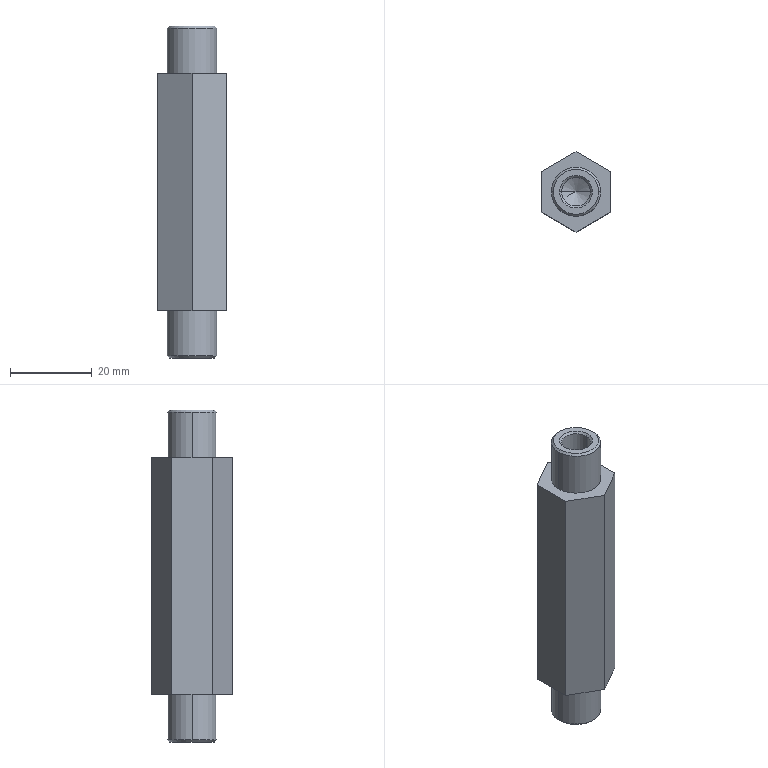Component | SolidWorks | YX-04-102GluePaperFeedingColumn-2 | 1 solid | 30 faces | box 17 x 19.63 x 81 mm | volume 15432 mm3 | cone 12 | plane 10 | cylinder 8 | commonest cylinder face diameters 7 x4 12 x4 | material Brass
build123d program:
from build123d import *

# Parameters (mm, degrees)
BOSS_EXTRUDE1_DEPTH          = 58
SKETCH2_W                    = 11.5
SKETCH2_H                    = 6
SKETCH3_W                    = 11.5
SKETCH3_H                    = 6
F_7_0_7_DIAMETER_HOLE1_D     = 7
F_7_0_7_DIAMETER_HOLE1_DEPTH = 21
F_7_0_7_DIAMETER_HOLE1_TIP   = 2.103
F_7_0_7_DIAMETER_HOLE2_D     = 7
F_7_0_7_DIAMETER_HOLE2_DEPTH = 21
F_7_0_7_DIAMETER_HOLE2_TIP   = 2.103
CHAMFER1_SIZE                = 0.5


with BuildPart() as part:
    # Sketch1 → Boss-Extrude1 (new body)
    with BuildSketch(Plane(origin=(29, 0, 0), x_dir=(0, 0, -1), z_dir=(1, 0, 0))):
        Polygon((8.5, -4.907), (8.5, 4.907), (0, 9.815), (-8.5, 4.907), (-8.5, -4.907), (0, -9.815), align=None)
    extrude(amount=-BOSS_EXTRUDE1_DEPTH)

    # Sketch2 → Revolve1 (revolve)
    with BuildSketch(Plane.XY, mode=Mode.PRIVATE) as revolve1_sk:
        with Locations((-34.75, 3)):
            Rectangle(SKETCH2_W, SKETCH2_H)
    revolve(revolve1_sk.sketch.rotate(Axis((-40.5, 0, 0), (1, 0, 0)), 270), axis=Axis((-40.5, 0, 0), (1, 0, 0)))

    # Sketch3 → Revolve2 (revolve)
    with BuildSketch(Plane.XY, mode=Mode.PRIVATE) as revolve2_sk:
        with Locations((34.75, 3)):
            Rectangle(SKETCH3_W, SKETCH3_H)
    revolve(revolve2_sk.sketch.rotate(Axis((29, 0, 0), (1, 0, 0)), 270), axis=Axis((29, 0, 0), (1, 0, 0)))

    # 7.0 _7_ Diameter Hole1
    with Locations(Plane.ZY.offset(40.5)):
        with Locations((0, 0)):
            Hole(F_7_0_7_DIAMETER_HOLE1_D / 2, depth=F_7_0_7_DIAMETER_HOLE1_DEPTH)
            with Locations((0, 0, -(F_7_0_7_DIAMETER_HOLE1_DEPTH + F_7_0_7_DIAMETER_HOLE1_TIP / 2))):  # 118° drill point
                Cone(0, F_7_0_7_DIAMETER_HOLE1_D / 2, F_7_0_7_DIAMETER_HOLE1_TIP, mode=Mode.SUBTRACT)

    # 7.0 _7_ Diameter Hole2
    with Locations(Plane(origin=(40.5, 0, 0), x_dir=(0, 0, -1), z_dir=(1, 0, 0))):
        with Locations((0, 0)):
            Hole(F_7_0_7_DIAMETER_HOLE2_D / 2, depth=F_7_0_7_DIAMETER_HOLE2_DEPTH)
            with Locations((0, 0, -(F_7_0_7_DIAMETER_HOLE2_DEPTH + F_7_0_7_DIAMETER_HOLE2_TIP / 2))):  # 118° drill point
                Cone(0, F_7_0_7_DIAMETER_HOLE2_D / 2, F_7_0_7_DIAMETER_HOLE2_TIP, mode=Mode.SUBTRACT)

    # Chamfer1
    chamfer1_edges = [part.edges().sort_by_distance(p)[0] for p in [
        (-40.5, 0, 6),
        (40.5, 0, 6),
        (-40.5, 0, 3.5),
        (40.5, 0, -3.5),
    ]]
    chamfer(chamfer1_edges, length=CHAMFER1_SIZE)


solid = part.part

# Placed as in the assembly
solid = solid.moved(Location((-123.397, 46.262, 235), (0, 90, 0)))
STEP:
#1=COLOUR_RGB('',0.7922,0.8196,0.9333);
#2=FILL_AREA_STYLE_COLOUR('',#1);
#3=FILL_AREA_STYLE('',(#2));
#4=SURFACE_STYLE_FILL_AREA(#3);
#5=SURFACE_SIDE_STYLE('',(#4));
#6=SURFACE_STYLE_USAGE(.BOTH.,#5);
#7=PRESENTATION_STYLE_ASSIGNMENT((#6));
#8=CARTESIAN_POINT('',(-4.72,1.821,7.677));
#9=VERTEX_POINT('',#8);
#10=CARTESIAN_POINT('',(-4.996,1.821,7.677));
#11=VERTEX_POINT('',#10);
#12=CARTESIAN_POINT('',(-4.858,1.821,7.677));
#13=DIRECTION('',(0.,0.,-1.));
#14=DIRECTION('',(-1.,0.,0.));
#15=AXIS2_PLACEMENT_3D('',#12,#13,#14);
#16=CIRCLE('',#15,0.1378);
#17=EDGE_CURVE('',#9,#11,#16,.T.);
#18=ORIENTED_EDGE('',*,*,#17,.F.);
#19=CARTESIAN_POINT('',(-4.701,1.821,7.657));
#20=VERTEX_POINT('',#19);
#21=CARTESIAN_POINT('',(-4.72,1.821,7.677));
#22=DIRECTION('',(0.7071,0.,-0.7071));
#23=VECTOR('',#22,39.37);
#24=LINE('',#21,#23);
#25=EDGE_CURVE('',#9,#20,#24,.T.);
#26=ORIENTED_EDGE('',*,*,#25,.T.);
#27=CARTESIAN_POINT('',(-5.016,1.821,7.657));
#28=VERTEX_POINT('',#27);
#29=CARTESIAN_POINT('',(-4.858,1.821,7.657));
#30=DIRECTION('',(0.,0.,1.));
#31=DIRECTION('',(-1.,0.,0.));
#32=AXIS2_PLACEMENT_3D('',#29,#30,#31);
#33=CIRCLE('',#32,0.1575);
#34=EDGE_CURVE('',#28,#20,#33,.T.);
#35=ORIENTED_EDGE('',*,*,#34,.F.);
#36=CARTESIAN_POINT('',(-4.996,1.821,7.677));
#37=DIRECTION('',(-0.7071,0.,-0.7071));
#38=VECTOR('',#37,39.37);
#39=LINE('',#36,#38);
#40=EDGE_CURVE('',#11,#28,#39,.T.);
#41=ORIENTED_EDGE('',*,*,#40,.F.);
#42=EDGE_LOOP('',(#18,#26,#35,#41));
#43=FACE_OUTER_BOUND('',#42,.T.);
#44=CARTESIAN_POINT('',(-4.858,1.821,7.677));
#45=DIRECTION('',(0.,0.,-1.));
#46=DIRECTION('',(-1.,0.,0.));
#47=AXIS2_PLACEMENT_3D('',#44,#45,#46);
#48=CONICAL_SURFACE('',#47,0.1378,0.7854);
#49=ADVANCED_FACE('',(#43),#48,.F.);
#50=CARTESIAN_POINT('',(-4.996,1.821,10.827));
#51=VERTEX_POINT('',#50);
#52=CARTESIAN_POINT('',(-4.72,1.821,10.827));
#53=VERTEX_POINT('',#52);
#54=CARTESIAN_POINT('',(-4.858,1.821,10.827));
#55=DIRECTION('',(0.,0.,1.));
#56=DIRECTION('',(1.,0.,0.));
#57=AXIS2_PLACEMENT_3D('',#54,#55,#56);
#58=CIRCLE('',#57,0.1378);
#59=EDGE_CURVE('',#51,#53,#58,.T.);
#60=ORIENTED_EDGE('',*,*,#59,.F.);
#61=CARTESIAN_POINT('',(-5.016,1.821,10.846));
#62=VERTEX_POINT('',#61);
#63=CARTESIAN_POINT('',(-4.996,1.821,10.827));
#64=DIRECTION('',(-0.7071,0.,0.7071));
#65=VECTOR('',#64,39.37);
#66=LINE('',#63,#65);
#67=EDGE_CURVE('',#51,#62,#66,.T.);
#68=ORIENTED_EDGE('',*,*,#67,.T.);
#69=CARTESIAN_POINT('',(-4.701,1.821,10.846));
#70=VERTEX_POINT('',#69);
#71=CARTESIAN_POINT('',(-4.858,1.821,10.846));
#72=DIRECTION('',(0.,0.,-1.));
#73=DIRECTION('',(1.,0.,0.));
#74=AXIS2_PLACEMENT_3D('',#71,#72,#73);
#75=CIRCLE('',#74,0.1575);
#76=EDGE_CURVE('',#70,#62,#75,.T.);
#77=ORIENTED_EDGE('',*,*,#76,.F.);
#78=CARTESIAN_POINT('',(-4.72,1.821,10.827));
#79=DIRECTION('',(0.7071,0.,0.7071));
#80=VECTOR('',#79,39.37);
#81=LINE('',#78,#80);
#82=EDGE_CURVE('',#53,#70,#81,.T.);
#83=ORIENTED_EDGE('',*,*,#82,.F.);
#84=EDGE_LOOP('',(#60,#68,#77,#83));
#85=FACE_OUTER_BOUND('',#84,.T.);
#86=CARTESIAN_POINT('',(-4.858,1.821,10.827));
#87=DIRECTION('',(0.,0.,1.));
#88=DIRECTION('',(1.,0.,0.));
#89=AXIS2_PLACEMENT_3D('',#86,#87,#88);
#90=CONICAL_SURFACE('',#89,0.1378,0.7854);
#91=ADVANCED_FACE('',(#85),#90,.F.);
#92=CARTESIAN_POINT('',(-4.642,1.821,10.846));
#93=VERTEX_POINT('',#92);
#94=CARTESIAN_POINT('',(-5.075,1.821,10.846));
#95=VERTEX_POINT('',#94);
#96=CARTESIAN_POINT('',(-4.858,1.821,10.846));
#97=DIRECTION('',(0.,0.,1.));
#98=DIRECTION('',(1.,0.,0.));
#99=AXIS2_PLACEMENT_3D('',#96,#97,#98);
#100=CIRCLE('',#99,0.2165);
#101=EDGE_CURVE('',#93,#95,#100,.T.);
#102=ORIENTED_EDGE('',*,*,#101,.F.);
#103=CARTESIAN_POINT('',(-4.622,1.821,10.827));
#104=VERTEX_POINT('',#103);
#105=CARTESIAN_POINT('',(-4.642,1.821,10.846));
#106=DIRECTION('',(0.7071,0.,-0.7071));
#107=VECTOR('',#106,39.37);
#108=LINE('',#105,#107);
#109=EDGE_CURVE('',#93,#104,#108,.T.);
#110=ORIENTED_EDGE('',*,*,#109,.T.);
#111=CARTESIAN_POINT('',(-5.094,1.821,10.827));
#112=VERTEX_POINT('',#111);
#113=CARTESIAN_POINT('',(-4.858,1.821,10.827));
#114=DIRECTION('',(0.,0.,-1.));
#115=DIRECTION('',(1.,0.,0.));
#116=AXIS2_PLACEMENT_3D('',#113,#114,#115);
#117=CIRCLE('',#116,0.2362);
#118=EDGE_CURVE('',#112,#104,#117,.T.);
#119=ORIENTED_EDGE('',*,*,#118,.F.);
#120=CARTESIAN_POINT('',(-5.075,1.821,10.846));
#121=DIRECTION('',(-0.7071,0.,-0.7071));
#122=VECTOR('',#121,39.37);
#123=LINE('',#120,#122);
#124=EDGE_CURVE('',#95,#112,#123,.T.);
#125=ORIENTED_EDGE('',*,*,#124,.F.);
#126=EDGE_LOOP('',(#102,#110,#119,#125));
#127=FACE_OUTER_BOUND('',#126,.T.);
#128=CARTESIAN_POINT('',(-4.858,1.821,10.846));
#129=DIRECTION('',(0.,0.,-1.));
#130=DIRECTION('',(-1.,0.,0.));
#131=AXIS2_PLACEMENT_3D('',#128,#129,#130);
#132=CONICAL_SURFACE('',#131,0.2165,0.7854);
#133=ADVANCED_FACE('',(#127),#132,.T.);
#134=CARTESIAN_POINT('',(-5.075,1.821,7.657));
#135=VERTEX_POINT('',#134);
#136=CARTESIAN_POINT('',(-4.642,1.821,7.657));
#137=VERTEX_POINT('',#136);
#138=CARTESIAN_POINT('',(-4.858,1.821,7.657));
#139=DIRECTION('',(0.,0.,-1.));
#140=DIRECTION('',(-1.,0.,0.));
#141=AXIS2_PLACEMENT_3D('',#138,#139,#140);
#142=CIRCLE('',#141,0.2165);
#143=EDGE_CURVE('',#135,#137,#142,.T.);
#144=ORIENTED_EDGE('',*,*,#143,.F.);
#145=CARTESIAN_POINT('',(-5.094,1.821,7.677));
#146=VERTEX_POINT('',#145);
#147=CARTESIAN_POINT('',(-5.094,1.821,7.677));
#148=DIRECTION('',(-0.7071,0.,0.7071));
#149=VECTOR('',#148,39.37);
#150=LINE('',#147,#149);
#151=EDGE_CURVE('',#135,#146,#150,.T.);
#152=ORIENTED_EDGE('',*,*,#151,.T.);
#153=CARTESIAN_POINT('',(-4.622,1.821,7.677));
#154=VERTEX_POINT('',#153);
#155=CARTESIAN_POINT('',(-4.858,1.821,7.677));
#156=DIRECTION('',(0.,0.,1.));
#157=DIRECTION('',(-1.,0.,0.));
#158=AXIS2_PLACEMENT_3D('',#155,#156,#157);
#159=CIRCLE('',#158,0.2362);
#160=EDGE_CURVE('',#154,#146,#159,.T.);
#161=ORIENTED_EDGE('',*,*,#160,.F.);
#162=CARTESIAN_POINT('',(-4.622,1.821,7.677));
#163=DIRECTION('',(0.7071,0.,0.7071));
#164=VECTOR('',#163,39.37);
#165=LINE('',#162,#164);
#166=EDGE_CURVE('',#137,#154,#165,.T.);
#167=ORIENTED_EDGE('',*,*,#166,.F.);
#168=EDGE_LOOP('',(#144,#152,#161,#167));
#169=FACE_OUTER_BOUND('',#168,.T.);
#170=CARTESIAN_POINT('',(-4.858,1.821,7.677));
#171=DIRECTION('',(0.,0.,1.));
#172=DIRECTION('',(1.,0.,0.));
#173=AXIS2_PLACEMENT_3D('',#170,#171,#172);
#174=CONICAL_SURFACE('',#173,0.2362,0.7854);
#175=ADVANCED_FACE('',(#169),#174,.T.);
#176=CARTESIAN_POINT('',(-4.996,1.821,10.02));
#177=VERTEX_POINT('',#176);
#178=CARTESIAN_POINT('',(-4.72,1.821,10.02));
#179=VERTEX_POINT('',#178);
#180=CARTESIAN_POINT('',(-4.858,1.821,10.02));
#181=DIRECTION('',(0.,0.,1.));
#182=DIRECTION('',(1.,0.,0.));
#183=AXIS2_PLACEMENT_3D('',#180,#181,#182);
#184=CIRCLE('',#183,0.1378);
#185=EDGE_CURVE('',#177,#179,#184,.T.);
#186=ORIENTED_EDGE('',*,*,#185,.F.);
#187=CARTESIAN_POINT('',(-4.996,1.821,10.846));
#188=DIRECTION('',(0.,0.,1.));
#189=VECTOR('',#188,39.37);
#190=LINE('',#187,#189);
#191=EDGE_CURVE('',#177,#51,#190,.T.);
#192=ORIENTED_EDGE('',*,*,#191,.T.);
#193=ORIENTED_EDGE('',*,*,#59,.T.);
#194=CARTESIAN_POINT('',(-4.72,1.821,10.846));
#195=DIRECTION('',(0.,0.,1.));
#196=VECTOR('',#195,39.37);
#197=LINE('',#194,#196);
#198=EDGE_CURVE('',#179,#53,#197,.T.);
#199=ORIENTED_EDGE('',*,*,#198,.F.);
#200=EDGE_LOOP('',(#186,#192,#193,#199));
#201=FACE_OUTER_BOUND('',#200,.T.);
#202=CARTESIAN_POINT('',(-4.858,1.821,10.846));
#203=DIRECTION('',(0.,0.,1.));
#204=DIRECTION('',(1.,0.,0.));
#205=AXIS2_PLACEMENT_3D('',#202,#203,#204);
#206=CYLINDRICAL_SURFACE('',#205,0.1378);
#207=ADVANCED_FACE('',(#201),#206,.F.);
#208=CARTESIAN_POINT('',(-4.858,1.821,9.937));
#209=VERTEX_POINT('',#208);
#210=CARTESIAN_POINT('',(-4.72,1.821,10.02));
#211=DIRECTION('',(0.8572,0.,0.515));
#212=VECTOR('',#211,39.37);
#213=LINE('',#210,#212);
#214=EDGE_CURVE('',#209,#179,#213,.T.);
#215=ORIENTED_EDGE('',*,*,#214,.F.);
#216=CARTESIAN_POINT('',(-4.996,1.821,10.02));
#217=DIRECTION('',(-0.8572,0.,0.515));
#218=VECTOR('',#217,39.37);
#219=LINE('',#216,#218);
#220=EDGE_CURVE('',#209,#177,#219,.T.);
#221=ORIENTED_EDGE('',*,*,#220,.T.);
#222=ORIENTED_EDGE('',*,*,#185,.T.);
#223=EDGE_LOOP('',(#215,#221,#222));
#224=FACE_OUTER_BOUND('',#223,.T.);
#225=CARTESIAN_POINT('',(-4.858,1.821,10.02));
#226=DIRECTION('',(0.,0.,1.));
#227=DIRECTION('',(1.,0.,0.));
#228=AXIS2_PLACEMENT_3D('',#225,#226,#227);
#229=CONICAL_SURFACE('',#228,0.1378,1.03);
#230=ADVANCED_FACE('',(#224),#229,.F.);
#231=CARTESIAN_POINT('',(-4.72,1.821,8.484));
#232=VERTEX_POINT('',#231);
#233=CARTESIAN_POINT('',(-4.996,1.821,8.484));
#234=VERTEX_POINT('',#233);
#235=CARTESIAN_POINT('',(-4.858,1.821,8.484));
#236=DIRECTION('',(0.,0.,-1.));
#237=DIRECTION('',(-1.,0.,0.));
#238=AXIS2_PLACEMENT_3D('',#235,#236,#237);
#239=CIRCLE('',#238,0.1378);
#240=EDGE_CURVE('',#232,#234,#239,.T.);
#241=ORIENTED_EDGE('',*,*,#240,.F.);
#242=CARTESIAN_POINT('',(-4.72,1.821,7.657));
#243=DIRECTION('',(0.,0.,-1.));
#244=VECTOR('',#243,39.37);
#245=LINE('',#242,#244);
#246=EDGE_CURVE('',#232,#9,#245,.T.);
#247=ORIENTED_EDGE('',*,*,#246,.T.);
#248=ORIENTED_EDGE('',*,*,#17,.T.);
#249=CARTESIAN_POINT('',(-4.996,1.821,7.657));
#250=DIRECTION('',(0.,0.,-1.));
#251=VECTOR('',#250,39.37);
#252=LINE('',#249,#251);
#253=EDGE_CURVE('',#234,#11,#252,.T.);
#254=ORIENTED_EDGE('',*,*,#253,.F.);
#255=EDGE_LOOP('',(#241,#247,#248,#254));
#256=FACE_OUTER_BOUND('',#255,.T.);
#257=CARTESIAN_POINT('',(-4.858,1.821,7.657));
#258=DIRECTION('',(0.,0.,-1.));
#259=DIRECTION('',(-1.,0.,0.));
#260=AXIS2_PLACEMENT_3D('',#257,#258,#259);
#261=CYLINDRICAL_SURFACE('',#260,0.1378);
#262=ADVANCED_FACE('',(#256),#261,.F.);
#263=CARTESIAN_POINT('',(-4.858,1.821,8.567));
#264=VERTEX_POINT('',#263);
#265=CARTESIAN_POINT('',(-4.996,1.821,8.484));
#266=DIRECTION('',(-0.8572,0.,-0.515));
#267=VECTOR('',#266,39.37);
#268=LINE('',#265,#267);
#269=EDGE_CURVE('',#264,#234,#268,.T.);
#270=ORIENTED_EDGE('',*,*,#269,.F.);
#271=CARTESIAN_POINT('',(-4.72,1.821,8.484));
#272=DIRECTION('',(0.8572,0.,-0.515));
#273=VECTOR('',#272,39.37);
#274=LINE('',#271,#273);
#275=EDGE_CURVE('',#264,#232,#274,.T.);
#276=ORIENTED_EDGE('',*,*,#275,.T.);
#277=ORIENTED_EDGE('',*,*,#240,.T.);
#278=EDGE_LOOP('',(#270,#276,#277));
#279=FACE_OUTER_BOUND('',#278,.T.);
#280=CARTESIAN_POINT('',(-4.858,1.821,8.484));
#281=DIRECTION('',(0.,0.,-1.));
#282=DIRECTION('',(-1.,0.,0.));
#283=AXIS2_PLACEMENT_3D('',#280,#281,#282);
#284=CONICAL_SURFACE('',#283,0.1378,1.03);
#285=ADVANCED_FACE('',(#279),#284,.F.);
#286=CARTESIAN_POINT('',(-4.622,1.821,10.394));
#287=VERTEX_POINT('',#286);
#288=CARTESIAN_POINT('',(-5.094,1.821,10.394));
#289=VERTEX_POINT('',#288);
#290=CARTESIAN_POINT('',(-4.858,1.821,10.394));
#291=DIRECTION('',(0.,0.,1.));
#292=DIRECTION('',(1.,0.,0.));
#293=AXIS2_PLACEMENT_3D('',#290,#291,#292);
#294=CIRCLE('',#293,0.2362);
#295=EDGE_CURVE('',#287,#289,#294,.T.);
#296=ORIENTED_EDGE('',*,*,#295,.T.);
#297=CARTESIAN_POINT('',(-5.094,1.821,10.394));
#298=DIRECTION('',(0.,0.,1.));
#299=VECTOR('',#298,39.37);
#300=LINE('',#297,#299);
#301=EDGE_CURVE('',#289,#112,#300,.T.);
#302=ORIENTED_EDGE('',*,*,#301,.T.);
#303=ORIENTED_EDGE('',*,*,#118,.T.);
#304=CARTESIAN_POINT('',(-4.622,1.821,10.394));
#305=DIRECTION('',(0.,0.,1.));
#306=VECTOR('',#305,39.37);
#307=LINE('',#304,#306);
#308=EDGE_CURVE('',#287,#104,#307,.T.);
#309=ORIENTED_EDGE('',*,*,#308,.F.);
#310=EDGE_LOOP('',(#296,#302,#303,#309));
#311=FACE_OUTER_BOUND('',#310,.T.);
#312=CARTESIAN_POINT('',(-4.858,1.821,10.394));
#313=DIRECTION('',(0.,0.,1.));
#314=DIRECTION('',(1.,0.,0.));
#315=AXIS2_PLACEMENT_3D('',#312,#313,#314);
#316=CYLINDRICAL_SURFACE('',#315,0.2362);
#317=ADVANCED_FACE('',(#311),#316,.T.);
#318=ORIENTED_EDGE('',*,*,#160,.T.);
#319=CARTESIAN_POINT('',(-5.094,1.821,8.11));
#320=VERTEX_POINT('',#319);
#321=CARTESIAN_POINT('',(-5.094,1.821,7.657));
#322=DIRECTION('',(0.,0.,1.));
#323=VECTOR('',#322,39.37);
#324=LINE('',#321,#323);
#325=EDGE_CURVE('',#146,#320,#324,.T.);
#326=ORIENTED_EDGE('',*,*,#325,.T.);
#327=CARTESIAN_POINT('',(-4.622,1.821,8.11));
#328=VERTEX_POINT('',#327);
#329=CARTESIAN_POINT('',(-4.858,1.821,8.11));
#330=DIRECTION('',(0.,0.,1.));
#331=DIRECTION('',(1.,0.,0.));
#332=AXIS2_PLACEMENT_3D('',#329,#330,#331);
#333=CIRCLE('',#332,0.2362);
#334=EDGE_CURVE('',#328,#320,#333,.T.);
#335=ORIENTED_EDGE('',*,*,#334,.F.);
#336=CARTESIAN_POINT('',(-4.622,1.821,7.657));
#337=DIRECTION('',(0.,0.,1.));
#338=VECTOR('',#337,39.37);
#339=LINE('',#336,#338);
#340=EDGE_CURVE('',#154,#328,#339,.T.);
#341=ORIENTED_EDGE('',*,*,#340,.F.);
#342=EDGE_LOOP('',(#318,#326,#335,#341));
#343=FACE_OUTER_BOUND('',#342,.T.);
#344=CARTESIAN_POINT('',(-4.858,1.821,7.657));
#345=DIRECTION('',(0.,0.,1.));
#346=DIRECTION('',(1.,0.,0.));
#347=AXIS2_PLACEMENT_3D('',#344,#345,#346);
#348=CYLINDRICAL_SURFACE('',#347,0.2362);
#349=ADVANCED_FACE('',(#343),#348,.T.);
#350=CARTESIAN_POINT('',(-4.858,1.435,10.394));
#351=VERTEX_POINT('',#350);
#352=CARTESIAN_POINT('',(-4.524,1.628,10.394));
#353=VERTEX_POINT('',#352);
#354=CARTESIAN_POINT('',(-4.858,1.435,10.394));
#355=DIRECTION('',(0.866,0.5,0.));
#356=VECTOR('',#355,39.37);
#357=LINE('',#354,#356);
#358=EDGE_CURVE('',#351,#353,#357,.T.);
#359=ORIENTED_EDGE('',*,*,#358,.F.);
#360=CARTESIAN_POINT('',(-4.858,1.435,8.11));
#361=VERTEX_POINT('',#360);
#362=CARTESIAN_POINT('',(-4.858,1.435,8.11));
#363=DIRECTION('',(0.,0.,1.));
#364=VECTOR('',#363,39.37);
#365=LINE('',#362,#364);
#366=EDGE_CURVE('',#361,#351,#365,.T.);
#367=ORIENTED_EDGE('',*,*,#366,.F.);
#368=CARTESIAN_POINT('',(-4.524,1.628,8.11));
#369=VERTEX_POINT('',#368);
#370=CARTESIAN_POINT('',(-4.858,1.435,8.11));
#371=DIRECTION('',(0.866,0.5,0.));
#372=VECTOR('',#371,39.37);
#373=LINE('',#370,#372);
#374=EDGE_CURVE('',#361,#369,#373,.T.);
#375=ORIENTED_EDGE('',*,*,#374,.T.);
#376=CARTESIAN_POINT('',(-4.524,1.628,8.11));
#377=DIRECTION('',(0.,0.,1.));
#378=VECTOR('',#377,39.37);
#379=LINE('',#376,#378);
#380=EDGE_CURVE('',#369,#353,#379,.T.);
#381=ORIENTED_EDGE('',*,*,#380,.T.);
#382=EDGE_LOOP('',(#359,#367,#375,#381));
#383=FACE_OUTER_BOUND('',#382,.T.);
#384=CARTESIAN_POINT('',(-4.858,1.435,8.11));
#385=DIRECTION('',(0.5,-0.866,0.));
#386=DIRECTION('',(0.866,0.5,0.));
#387=AXIS2_PLACEMENT_3D('',#384,#385,#386);
#388=PLANE('',#387);
#389=ADVANCED_FACE('',(#383),#388,.T.);
#390=CARTESIAN_POINT('',(-5.193,1.628,10.394));
#391=VERTEX_POINT('',#390);
#392=CARTESIAN_POINT('',(-5.193,1.628,10.394));
#393=DIRECTION('',(0.866,-0.5,0.));
#394=VECTOR('',#393,39.37);
#395=LINE('',#392,#394);
#396=EDGE_CURVE('',#391,#351,#395,.T.);
#397=ORIENTED_EDGE('',*,*,#396,.F.);
#398=CARTESIAN_POINT('',(-5.193,1.628,8.11));
#399=VERTEX_POINT('',#398);
#400=CARTESIAN_POINT('',(-5.193,1.628,8.11));
#401=DIRECTION('',(0.,0.,1.));
#402=VECTOR('',#401,39.37);
#403=LINE('',#400,#402);
#404=EDGE_CURVE('',#399,#391,#403,.T.);
#405=ORIENTED_EDGE('',*,*,#404,.F.);
#406=CARTESIAN_POINT('',(-5.193,1.628,8.11));
#407=DIRECTION('',(0.866,-0.5,0.));
#408=VECTOR('',#407,39.37);
#409=LINE('',#406,#408);
#410=EDGE_CURVE('',#399,#361,#409,.T.);
#411=ORIENTED_EDGE('',*,*,#410,.T.);
#412=ORIENTED_EDGE('',*,*,#366,.T.);
#413=EDGE_LOOP('',(#397,#405,#411,#412));
#414=FACE_OUTER_BOUND('',#413,.T.);
#415=CARTESIAN_POINT('',(-5.193,1.628,8.11));
#416=DIRECTION('',(-0.5,-0.866,0.));
#417=DIRECTION('',(0.866,-0.5,0.));
#418=AXIS2_PLACEMENT_3D('',#415,#416,#417);
#419=PLANE('',#418);
#420=ADVANCED_FACE('',(#414),#419,.T.);
#421=CARTESIAN_POINT('',(-5.193,2.015,10.394));
#422=VERTEX_POINT('',#421);
#423=CARTESIAN_POINT('',(-5.193,2.015,10.394));
#424=DIRECTION('',(-0.,-1.,0.));
#425=VECTOR('',#424,39.37);
#426=LINE('',#423,#425);
#427=EDGE_CURVE('',#422,#391,#426,.T.);
#428=ORIENTED_EDGE('',*,*,#427,.F.);
#429=CARTESIAN_POINT('',(-5.193,2.015,8.11));
#430=VERTEX_POINT('',#429);
#431=CARTESIAN_POINT('',(-5.193,2.015,8.11));
#432=DIRECTION('',(0.,0.,1.));
#433=VECTOR('',#432,39.37);
#434=LINE('',#431,#433);
#435=EDGE_CURVE('',#430,#422,#434,.T.);
#436=ORIENTED_EDGE('',*,*,#435,.F.);
#437=CARTESIAN_POINT('',(-5.193,2.015,8.11));
#438=DIRECTION('',(-0.,-1.,0.));
#439=VECTOR('',#438,39.37);
#440=LINE('',#437,#439);
#441=EDGE_CURVE('',#430,#399,#440,.T.);
#442=ORIENTED_EDGE('',*,*,#441,.T.);
#443=ORIENTED_EDGE('',*,*,#404,.T.);
#444=EDGE_LOOP('',(#428,#436,#442,#443));
#445=FACE_OUTER_BOUND('',#444,.T.);
#446=CARTESIAN_POINT('',(-5.193,2.015,8.11));
#447=DIRECTION('',(-1.,0.,0.));
#448=DIRECTION('',(-0.,-1.,0.));
#449=AXIS2_PLACEMENT_3D('',#446,#447,#448);
#450=PLANE('',#449);
#451=ADVANCED_FACE('',(#445),#450,.T.);
#452=CARTESIAN_POINT('',(-4.858,2.208,10.394));
#453=VERTEX_POINT('',#452);
#454=CARTESIAN_POINT('',(-4.858,2.208,10.394));
#455=DIRECTION('',(-0.866,-0.5,0.));
#456=VECTOR('',#455,39.37);
#457=LINE('',#454,#456);
#458=EDGE_CURVE('',#453,#422,#457,.T.);
#459=ORIENTED_EDGE('',*,*,#458,.F.);
#460=CARTESIAN_POINT('',(-4.858,2.208,8.11));
#461=VERTEX_POINT('',#460);
#462=CARTESIAN_POINT('',(-4.858,2.208,8.11));
#463=DIRECTION('',(0.,0.,1.));
#464=VECTOR('',#463,39.37);
#465=LINE('',#462,#464);
#466=EDGE_CURVE('',#461,#453,#465,.T.);
#467=ORIENTED_EDGE('',*,*,#466,.F.);
#468=CARTESIAN_POINT('',(-4.858,2.208,8.11));
#469=DIRECTION('',(-0.866,-0.5,0.));
#470=VECTOR('',#469,39.37);
#471=LINE('',#468,#470);
#472=EDGE_CURVE('',#461,#430,#471,.T.);
#473=ORIENTED_EDGE('',*,*,#472,.T.);
#474=ORIENTED_EDGE('',*,*,#435,.T.);
#475=EDGE_LOOP('',(#459,#467,#473,#474));
#476=FACE_OUTER_BOUND('',#475,.T.);
#477=CARTESIAN_POINT('',(-4.858,2.208,8.11));
#478=DIRECTION('',(-0.5,0.866,0.));
#479=DIRECTION('',(-0.866,-0.5,0.));
#480=AXIS2_PLACEMENT_3D('',#477,#478,#479);
#481=PLANE('',#480);
#482=ADVANCED_FACE('',(#476),#481,.T.);
#483=CARTESIAN_POINT('',(-4.524,2.015,10.394));
#484=VERTEX_POINT('',#483);
#485=CARTESIAN_POINT('',(-4.524,2.015,10.394));
#486=DIRECTION('',(-0.866,0.5,0.));
#487=VECTOR('',#486,39.37);
#488=LINE('',#485,#487);
#489=EDGE_CURVE('',#484,#453,#488,.T.);
#490=ORIENTED_EDGE('',*,*,#489,.F.);
#491=CARTESIAN_POINT('',(-4.524,2.015,8.11));
#492=VERTEX_POINT('',#491);
#493=CARTESIAN_POINT('',(-4.524,2.015,8.11));
#494=DIRECTION('',(0.,0.,1.));
#495=VECTOR('',#494,39.37);
#496=LINE('',#493,#495);
#497=EDGE_CURVE('',#492,#484,#496,.T.);
#498=ORIENTED_EDGE('',*,*,#497,.F.);
#499=CARTESIAN_POINT('',(-4.524,2.015,8.11));
#500=DIRECTION('',(-0.866,0.5,0.));
#501=VECTOR('',#500,39.37);
#502=LINE('',#499,#501);
#503=EDGE_CURVE('',#492,#461,#502,.T.);
#504=ORIENTED_EDGE('',*,*,#503,.T.);
#505=ORIENTED_EDGE('',*,*,#466,.T.);
#506=EDGE_LOOP('',(#490,#498,#504,#505));
#507=FACE_OUTER_BOUND('',#506,.T.);
#508=CARTESIAN_POINT('',(-4.524,2.015,8.11));
#509=DIRECTION('',(0.5,0.866,0.));
#510=DIRECTION('',(-0.866,0.5,0.));
#511=AXIS2_PLACEMENT_3D('',#508,#509,#510);
#512=PLANE('',#511);
#513=ADVANCED_FACE('',(#507),#512,.T.);
#514=CARTESIAN_POINT('',(-4.524,1.628,10.394));
#515=DIRECTION('',(0.,1.,0.));
#516=VECTOR('',#515,39.37);
#517=LINE('',#514,#516);
#518=EDGE_CURVE('',#353,#484,#517,.T.);
#519=ORIENTED_EDGE('',*,*,#518,.F.);
#520=ORIENTED_EDGE('',*,*,#380,.F.);
#521=CARTESIAN_POINT('',(-4.524,1.628,8.11));
#522=DIRECTION('',(0.,1.,0.));
#523=VECTOR('',#522,39.37);
#524=LINE('',#521,#523);
#525=EDGE_CURVE('',#369,#492,#524,.T.);
#526=ORIENTED_EDGE('',*,*,#525,.T.);
#527=ORIENTED_EDGE('',*,*,#497,.T.);
#528=EDGE_LOOP('',(#519,#520,#526,#527));
#529=FACE_OUTER_BOUND('',#528,.T.);
#530=CARTESIAN_POINT('',(-4.524,1.628,8.11));
#531=DIRECTION('',(1.,-0.,0.));
#532=DIRECTION('',(0.,1.,0.));
#533=AXIS2_PLACEMENT_3D('',#530,#531,#532);
#534=PLANE('',#533);
#535=ADVANCED_FACE('',(#529),#534,.T.);
#536=ORIENTED_EDGE('',*,*,#334,.T.);
#537=CARTESIAN_POINT('',(-4.858,1.821,8.11));
#538=DIRECTION('',(0.,0.,1.));
#539=DIRECTION('',(1.,0.,0.));
#540=AXIS2_PLACEMENT_3D('',#537,#538,#539);
#541=CIRCLE('',#540,0.2362);
#542=EDGE_CURVE('',#320,#328,#541,.T.);
#543=ORIENTED_EDGE('',*,*,#542,.T.);
#544=EDGE_LOOP('',(#536,#543));
#545=FACE_BOUND('',#544,.T.);
#546=ORIENTED_EDGE('',*,*,#374,.F.);
#547=ORIENTED_EDGE('',*,*,#410,.F.);
#548=ORIENTED_EDGE('',*,*,#441,.F.);
#549=ORIENTED_EDGE('',*,*,#472,.F.);
#550=ORIENTED_EDGE('',*,*,#503,.F.);
#551=ORIENTED_EDGE('',*,*,#525,.F.);
#552=EDGE_LOOP('',(#546,#547,#548,#549,#550,#551));
#553=FACE_OUTER_BOUND('',#552,.T.);
#554=CARTESIAN_POINT('',(-4.858,1.821,8.11));
#555=DIRECTION('',(0.,0.,1.));
#556=DIRECTION('',(1.,0.,0.));
#557=AXIS2_PLACEMENT_3D('',#554,#555,#556);
#558=PLANE('',#557);
#559=ADVANCED_FACE('',(#545,#553),#558,.F.);
#560=ORIENTED_EDGE('',*,*,#295,.F.);
#561=CARTESIAN_POINT('',(-4.858,1.821,10.394));
#562=DIRECTION('',(0.,0.,1.));
#563=DIRECTION('',(1.,0.,0.));
#564=AXIS2_PLACEMENT_3D('',#561,#562,#563);
#565=CIRCLE('',#564,0.2362);
#566=EDGE_CURVE('',#289,#287,#565,.T.);
#567=ORIENTED_EDGE('',*,*,#566,.F.);
#568=EDGE_LOOP('',(#560,#567));
#569=FACE_BOUND('',#568,.T.);
#570=ORIENTED_EDGE('',*,*,#358,.T.);
#571=ORIENTED_EDGE('',*,*,#518,.T.);
#572=ORIENTED_EDGE('',*,*,#489,.T.);
#573=ORIENTED_EDGE('',*,*,#458,.T.);
#574=ORIENTED_EDGE('',*,*,#427,.T.);
#575=ORIENTED_EDGE('',*,*,#396,.T.);
#576=EDGE_LOOP('',(#570,#571,#572,#573,#574,#575));
#577=FACE_OUTER_BOUND('',#576,.T.);
#578=CARTESIAN_POINT('',(-4.858,1.821,10.394));
#579=DIRECTION('',(0.,0.,1.));
#580=DIRECTION('',(1.,0.,0.));
#581=AXIS2_PLACEMENT_3D('',#578,#579,#580);
#582=PLANE('',#581);
#583=ADVANCED_FACE('',(#569,#577),#582,.T.);
#584=ORIENTED_EDGE('',*,*,#325,.F.);
#585=CARTESIAN_POINT('',(-4.858,1.821,7.677));
#586=DIRECTION('',(0.,0.,1.));
#587=DIRECTION('',(-1.,0.,0.));
#588=AXIS2_PLACEMENT_3D('',#585,#586,#587);
#589=CIRCLE('',#588,0.2362);
#590=EDGE_CURVE('',#146,#154,#589,.T.);
#591=ORIENTED_EDGE('',*,*,#590,.T.);
#592=ORIENTED_EDGE('',*,*,#340,.T.);
#593=ORIENTED_EDGE('',*,*,#542,.F.);
#594=EDGE_LOOP('',(#584,#591,#592,#593));
#595=FACE_OUTER_BOUND('',#594,.T.);
#596=CARTESIAN_POINT('',(-4.858,1.821,7.657));
#597=DIRECTION('',(0.,0.,1.));
#598=DIRECTION('',(1.,0.,0.));
#599=AXIS2_PLACEMENT_3D('',#596,#597,#598);
#600=CYLINDRICAL_SURFACE('',#599,0.2362);
#601=ADVANCED_FACE('',(#595),#600,.T.);
#602=CARTESIAN_POINT('',(-4.858,1.821,7.657));
#603=DIRECTION('',(0.,0.,-1.));
#604=DIRECTION('',(-1.,0.,0.));
#605=AXIS2_PLACEMENT_3D('',#602,#603,#604);
#606=CIRCLE('',#605,0.2165);
#607=EDGE_CURVE('',#137,#135,#606,.T.);
#608=ORIENTED_EDGE('',*,*,#607,.T.);
#609=ORIENTED_EDGE('',*,*,#143,.T.);
#610=EDGE_LOOP('',(#608,#609));
#611=FACE_OUTER_BOUND('',#610,.T.);
#612=ORIENTED_EDGE('',*,*,#34,.T.);
#613=CARTESIAN_POINT('',(-4.858,1.821,7.657));
#614=DIRECTION('',(0.,0.,1.));
#615=DIRECTION('',(-1.,0.,0.));
#616=AXIS2_PLACEMENT_3D('',#613,#614,#615);
#617=CIRCLE('',#616,0.1575);
#618=EDGE_CURVE('',#20,#28,#617,.T.);
#619=ORIENTED_EDGE('',*,*,#618,.T.);
#620=EDGE_LOOP('',(#612,#619));
#621=FACE_BOUND('',#620,.T.);
#622=CARTESIAN_POINT('',(-4.858,2.058,7.657));
#623=DIRECTION('',(0.,0.,-1.));
#624=DIRECTION('',(-1.,0.,0.));
#625=AXIS2_PLACEMENT_3D('',#622,#623,#624);
#626=PLANE('',#625);
#627=ADVANCED_FACE('',(#611,#621),#626,.T.);
#628=ORIENTED_EDGE('',*,*,#301,.F.);
#629=ORIENTED_EDGE('',*,*,#566,.T.);
#630=ORIENTED_EDGE('',*,*,#308,.T.);
#631=CARTESIAN_POINT('',(-4.858,1.821,10.827));
#632=DIRECTION('',(0.,0.,-1.));
#633=DIRECTION('',(1.,0.,0.));
#634=AXIS2_PLACEMENT_3D('',#631,#632,#633);
#635=CIRCLE('',#634,0.2362);
#636=EDGE_CURVE('',#104,#112,#635,.T.);
#637=ORIENTED_EDGE('',*,*,#636,.T.);
#638=EDGE_LOOP('',(#628,#629,#630,#637));
#639=FACE_OUTER_BOUND('',#638,.T.);
#640=CARTESIAN_POINT('',(-4.858,1.821,10.394));
#641=DIRECTION('',(0.,0.,1.));
#642=DIRECTION('',(1.,0.,0.));
#643=AXIS2_PLACEMENT_3D('',#640,#641,#642);
#644=CYLINDRICAL_SURFACE('',#643,0.2362);
#645=ADVANCED_FACE('',(#639),#644,.T.);
#646=CARTESIAN_POINT('',(-4.858,1.821,10.846));
#647=DIRECTION('',(0.,0.,1.));
#648=DIRECTION('',(1.,0.,0.));
#649=AXIS2_PLACEMENT_3D('',#646,#647,#648);
#650=CIRCLE('',#649,0.2165);
#651=EDGE_CURVE('',#95,#93,#650,.T.);
#652=ORIENTED_EDGE('',*,*,#651,.T.);
#653=ORIENTED_EDGE('',*,*,#101,.T.);
#654=EDGE_LOOP('',(#652,#653));
#655=FACE_OUTER_BOUND('',#654,.T.);
#656=ORIENTED_EDGE('',*,*,#76,.T.);
#657=CARTESIAN_POINT('',(-4.858,1.821,10.846));
#658=DIRECTION('',(0.,0.,-1.));
#659=DIRECTION('',(1.,0.,0.));
#660=AXIS2_PLACEMENT_3D('',#657,#658,#659);
#661=CIRCLE('',#660,0.1575);
#662=EDGE_CURVE('',#62,#70,#661,.T.);
#663=ORIENTED_EDGE('',*,*,#662,.T.);
#664=EDGE_LOOP('',(#656,#663));
#665=FACE_BOUND('',#664,.T.);
#666=CARTESIAN_POINT('',(-4.858,1.821,10.846));
#667=DIRECTION('',(0.,0.,1.));
#668=DIRECTION('',(1.,0.,0.));
#669=AXIS2_PLACEMENT_3D('',#666,#667,#668);
#670=PLANE('',#669);
#671=ADVANCED_FACE('',(#655,#665),#670,.T.);
#672=ORIENTED_EDGE('',*,*,#275,.F.);
#673=ORIENTED_EDGE('',*,*,#269,.T.);
#674=CARTESIAN_POINT('',(-4.858,1.821,8.484));
#675=DIRECTION('',(0.,0.,-1.));
#676=DIRECTION('',(-1.,0.,0.));
#677=AXIS2_PLACEMENT_3D('',#674,#675,#676);
#678=CIRCLE('',#677,0.1378);
#679=EDGE_CURVE('',#234,#232,#678,.T.);
#680=ORIENTED_EDGE('',*,*,#679,.T.);
#681=EDGE_LOOP('',(#672,#673,#680));
#682=FACE_OUTER_BOUND('',#681,.T.);
#683=CARTESIAN_POINT('',(-4.858,1.821,8.484));
#684=DIRECTION('',(0.,0.,-1.));
#685=DIRECTION('',(-1.,0.,0.));
#686=AXIS2_PLACEMENT_3D('',#683,#684,#685);
#687=CONICAL_SURFACE('',#686,0.1378,1.03);
#688=ADVANCED_FACE('',(#682),#687,.F.);
#689=ORIENTED_EDGE('',*,*,#246,.F.);
#690=ORIENTED_EDGE('',*,*,#679,.F.);
#691=ORIENTED_EDGE('',*,*,#253,.T.);
#692=CARTESIAN_POINT('',(-4.858,1.821,7.677));
#693=DIRECTION('',(0.,0.,-1.));
#694=DIRECTION('',(-1.,0.,0.));
#695=AXIS2_PLACEMENT_3D('',#692,#693,#694);
#696=CIRCLE('',#695,0.1378);
#697=EDGE_CURVE('',#11,#9,#696,.T.);
#698=ORIENTED_EDGE('',*,*,#697,.T.);
#699=EDGE_LOOP('',(#689,#690,#691,#698));
#700=FACE_OUTER_BOUND('',#699,.T.);
#701=CARTESIAN_POINT('',(-4.858,1.821,7.657));
#702=DIRECTION('',(0.,0.,-1.));
#703=DIRECTION('',(-1.,0.,0.));
#704=AXIS2_PLACEMENT_3D('',#701,#702,#703);
#705=CYLINDRICAL_SURFACE('',#704,0.1378);
#706=ADVANCED_FACE('',(#700),#705,.F.);
#707=ORIENTED_EDGE('',*,*,#220,.F.);
#708=ORIENTED_EDGE('',*,*,#214,.T.);
#709=CARTESIAN_POINT('',(-4.858,1.821,10.02));
#710=DIRECTION('',(0.,0.,1.));
#711=DIRECTION('',(1.,0.,0.));
#712=AXIS2_PLACEMENT_3D('',#709,#710,#711);
#713=CIRCLE('',#712,0.1378);
#714=EDGE_CURVE('',#179,#177,#713,.T.);
#715=ORIENTED_EDGE('',*,*,#714,.T.);
#716=EDGE_LOOP('',(#707,#708,#715));
#717=FACE_OUTER_BOUND('',#716,.T.);
#718=CARTESIAN_POINT('',(-4.858,1.821,10.02));
#719=DIRECTION('',(0.,0.,1.));
#720=DIRECTION('',(1.,0.,0.));
#721=AXIS2_PLACEMENT_3D('',#718,#719,#720);
#722=CONICAL_SURFACE('',#721,0.1378,1.03);
#723=ADVANCED_FACE('',(#717),#722,.F.);
#724=ORIENTED_EDGE('',*,*,#191,.F.);
#725=ORIENTED_EDGE('',*,*,#714,.F.);
#726=ORIENTED_EDGE('',*,*,#198,.T.);
#727=CARTESIAN_POINT('',(-4.858,1.821,10.827));
#728=DIRECTION('',(0.,0.,1.));
#729=DIRECTION('',(1.,0.,0.));
#730=AXIS2_PLACEMENT_3D('',#727,#728,#729);
#731=CIRCLE('',#730,0.1378);
#732=EDGE_CURVE('',#53,#51,#731,.T.);
#733=ORIENTED_EDGE('',*,*,#732,.T.);
#734=EDGE_LOOP('',(#724,#725,#726,#733));
#735=FACE_OUTER_BOUND('',#734,.T.);
#736=CARTESIAN_POINT('',(-4.858,1.821,10.846));
#737=DIRECTION('',(0.,0.,1.));
#738=DIRECTION('',(1.,0.,0.));
#739=AXIS2_PLACEMENT_3D('',#736,#737,#738);
#740=CYLINDRICAL_SURFACE('',#739,0.1378);
#741=ADVANCED_FACE('',(#735),#740,.F.);
#742=ORIENTED_EDGE('',*,*,#151,.F.);
#743=ORIENTED_EDGE('',*,*,#607,.F.);
#744=ORIENTED_EDGE('',*,*,#166,.T.);
#745=ORIENTED_EDGE('',*,*,#590,.F.);
#746=EDGE_LOOP('',(#742,#743,#744,#745));
#747=FACE_OUTER_BOUND('',#746,.T.);
#748=CARTESIAN_POINT('',(-4.858,1.821,7.677));
#749=DIRECTION('',(0.,0.,1.));
#750=DIRECTION('',(1.,0.,0.));
#751=AXIS2_PLACEMENT_3D('',#748,#749,#750);
#752=CONICAL_SURFACE('',#751,0.2362,0.7854);
#753=ADVANCED_FACE('',(#747),#752,.T.);
#754=ORIENTED_EDGE('',*,*,#109,.F.);
#755=ORIENTED_EDGE('',*,*,#651,.F.);
#756=ORIENTED_EDGE('',*,*,#124,.T.);
#757=ORIENTED_EDGE('',*,*,#636,.F.);
#758=EDGE_LOOP('',(#754,#755,#756,#757));
#759=FACE_OUTER_BOUND('',#758,.T.);
#760=CARTESIAN_POINT('',(-4.858,1.821,10.846));
#761=DIRECTION('',(0.,0.,-1.));
#762=DIRECTION('',(-1.,0.,0.));
#763=AXIS2_PLACEMENT_3D('',#760,#761,#762);
#764=CONICAL_SURFACE('',#763,0.2165,0.7854);
#765=ADVANCED_FACE('',(#759),#764,.T.);
#766=ORIENTED_EDGE('',*,*,#67,.F.);
#767=ORIENTED_EDGE('',*,*,#732,.F.);
#768=ORIENTED_EDGE('',*,*,#82,.T.);
#769=ORIENTED_EDGE('',*,*,#662,.F.);
#770=EDGE_LOOP('',(#766,#767,#768,#769));
#771=FACE_OUTER_BOUND('',#770,.T.);
#772=CARTESIAN_POINT('',(-4.858,1.821,10.827));
#773=DIRECTION('',(0.,0.,1.));
#774=DIRECTION('',(1.,0.,0.));
#775=AXIS2_PLACEMENT_3D('',#772,#773,#774);
#776=CONICAL_SURFACE('',#775,0.1378,0.7854);
#777=ADVANCED_FACE('',(#771),#776,.F.);
#778=ORIENTED_EDGE('',*,*,#25,.F.);
#779=ORIENTED_EDGE('',*,*,#697,.F.);
#780=ORIENTED_EDGE('',*,*,#40,.T.);
#781=ORIENTED_EDGE('',*,*,#618,.F.);
#782=EDGE_LOOP('',(#778,#779,#780,#781));
#783=FACE_OUTER_BOUND('',#782,.T.);
#784=CARTESIAN_POINT('',(-4.858,1.821,7.677));
#785=DIRECTION('',(0.,0.,-1.));
#786=DIRECTION('',(-1.,0.,0.));
#787=AXIS2_PLACEMENT_3D('',#784,#785,#786);
#788=CONICAL_SURFACE('',#787,0.1378,0.7854);
#789=ADVANCED_FACE('',(#783),#788,.F.);
#790=CLOSED_SHELL('',(#49,#91,#133,#175,#207,#230,#262,#285,#317,#349,#389,#420,#451,#482,#513,#535,#559,#583,#601,#627,#645,#671,#688,#706,#723,#741,#753,#765,#777,#789));
#791=MANIFOLD_SOLID_BREP('',#790);
#792=STYLED_ITEM('',(#7),#791);
#793=(LENGTH_UNIT()NAMED_UNIT(*)SI_UNIT($,.METRE.));
#794=LENGTH_MEASURE_WITH_UNIT(LENGTH_MEASURE(0.0254),#793);
#795=DIMENSIONAL_EXPONENTS(1.,0.,0.,0.,0.,0.,0.);
#796=(CONVERSION_BASED_UNIT('',#794)LENGTH_UNIT()NAMED_UNIT(#795));
#797=UNCERTAINTY_MEASURE_WITH_UNIT(LENGTH_MEASURE(0.00001),#796,'','');
#798=(NAMED_UNIT(*)PLANE_ANGLE_UNIT()SI_UNIT($,.RADIAN.));
#799=(NAMED_UNIT(*)SI_UNIT($,.STERADIAN.)SOLID_ANGLE_UNIT());
#800=(GEOMETRIC_REPRESENTATION_CONTEXT(3)GLOBAL_UNCERTAINTY_ASSIGNED_CONTEXT((#797))GLOBAL_UNIT_ASSIGNED_CONTEXT((#796,#798,#799))REPRESENTATION_CONTEXT('',''));
#801=MECHANICAL_DESIGN_GEOMETRIC_PRESENTATION_REPRESENTATION('',(#792),#800);
#802=CARTESIAN_POINT('',(0.,0.,0.));
#803=DIRECTION('',(0.,0.,1.));
#804=DIRECTION('',(1.,0.,0.));
#805=AXIS2_PLACEMENT_3D('',#802,#803,#804);
#806=(LENGTH_UNIT()NAMED_UNIT(*)SI_UNIT($,.METRE.));
#807=LENGTH_MEASURE_WITH_UNIT(LENGTH_MEASURE(0.0254),#806);
#808=DIMENSIONAL_EXPONENTS(1.,0.,0.,0.,0.,0.,0.);
#809=(CONVERSION_BASED_UNIT('',#807)LENGTH_UNIT()NAMED_UNIT(#808));
#810=UNCERTAINTY_MEASURE_WITH_UNIT(LENGTH_MEASURE(0.00001),#809,'','');
#811=(NAMED_UNIT(*)PLANE_ANGLE_UNIT()SI_UNIT($,.RADIAN.));
#812=(NAMED_UNIT(*)SI_UNIT($,.STERADIAN.)SOLID_ANGLE_UNIT());
#813=(GEOMETRIC_REPRESENTATION_CONTEXT(3)GLOBAL_UNCERTAINTY_ASSIGNED_CONTEXT((#810))GLOBAL_UNIT_ASSIGNED_CONTEXT((#809,#811,#812))REPRESENTATION_CONTEXT('',''));
#814=ADVANCED_BREP_SHAPE_REPRESENTATION('',(#791,#805),#813);
#815=PRESENTATION_LAYER_ASSIGNMENT('','',(#792));